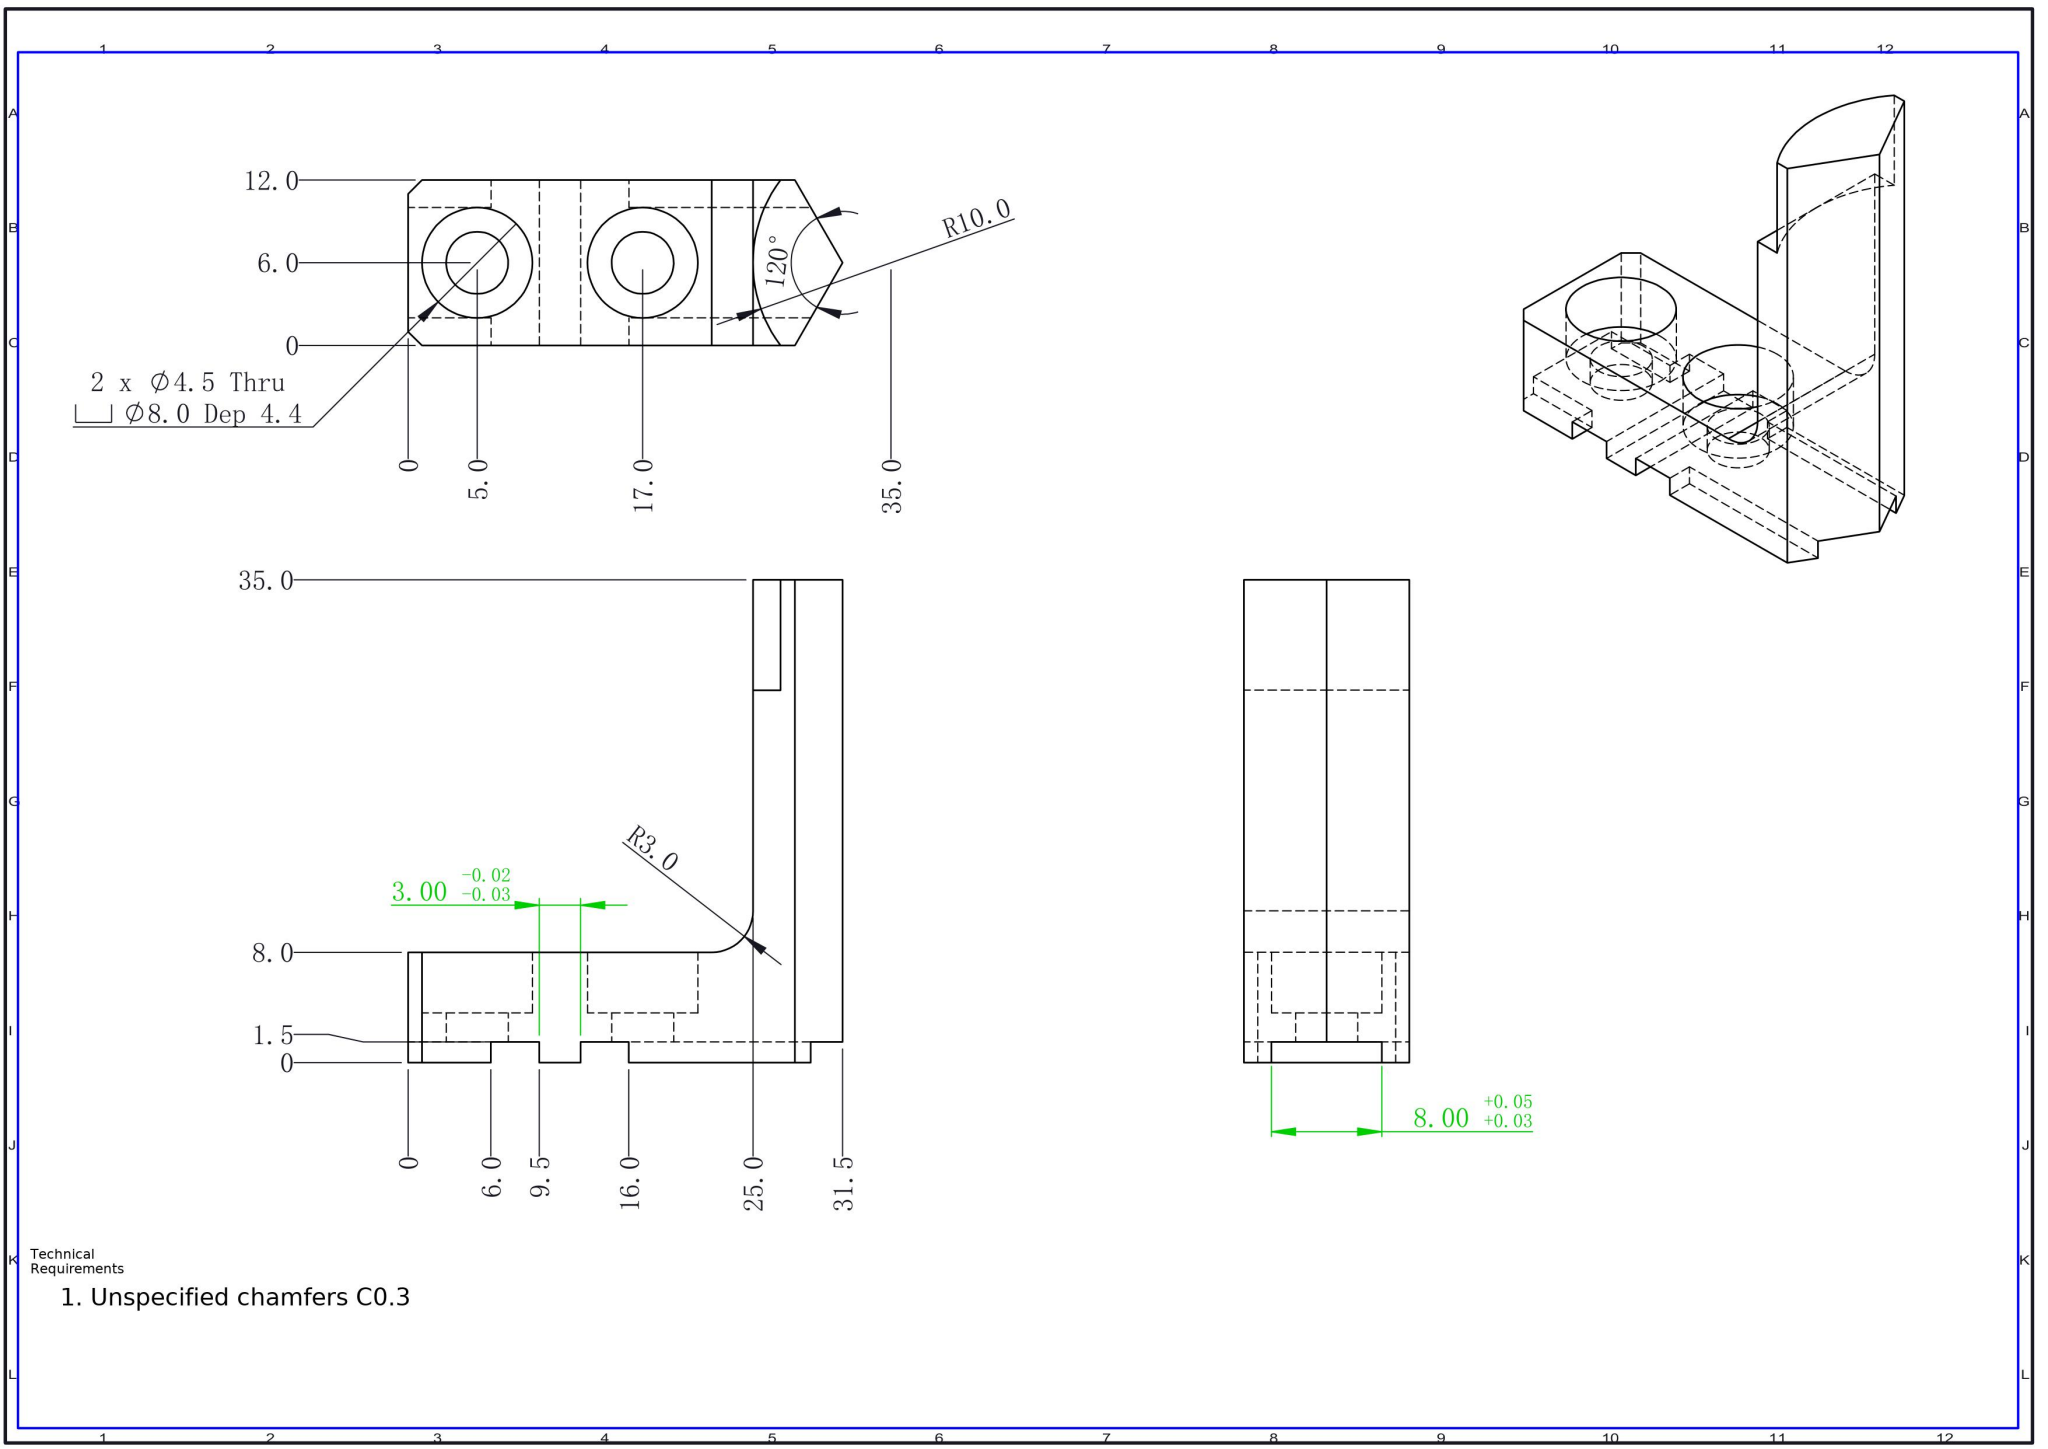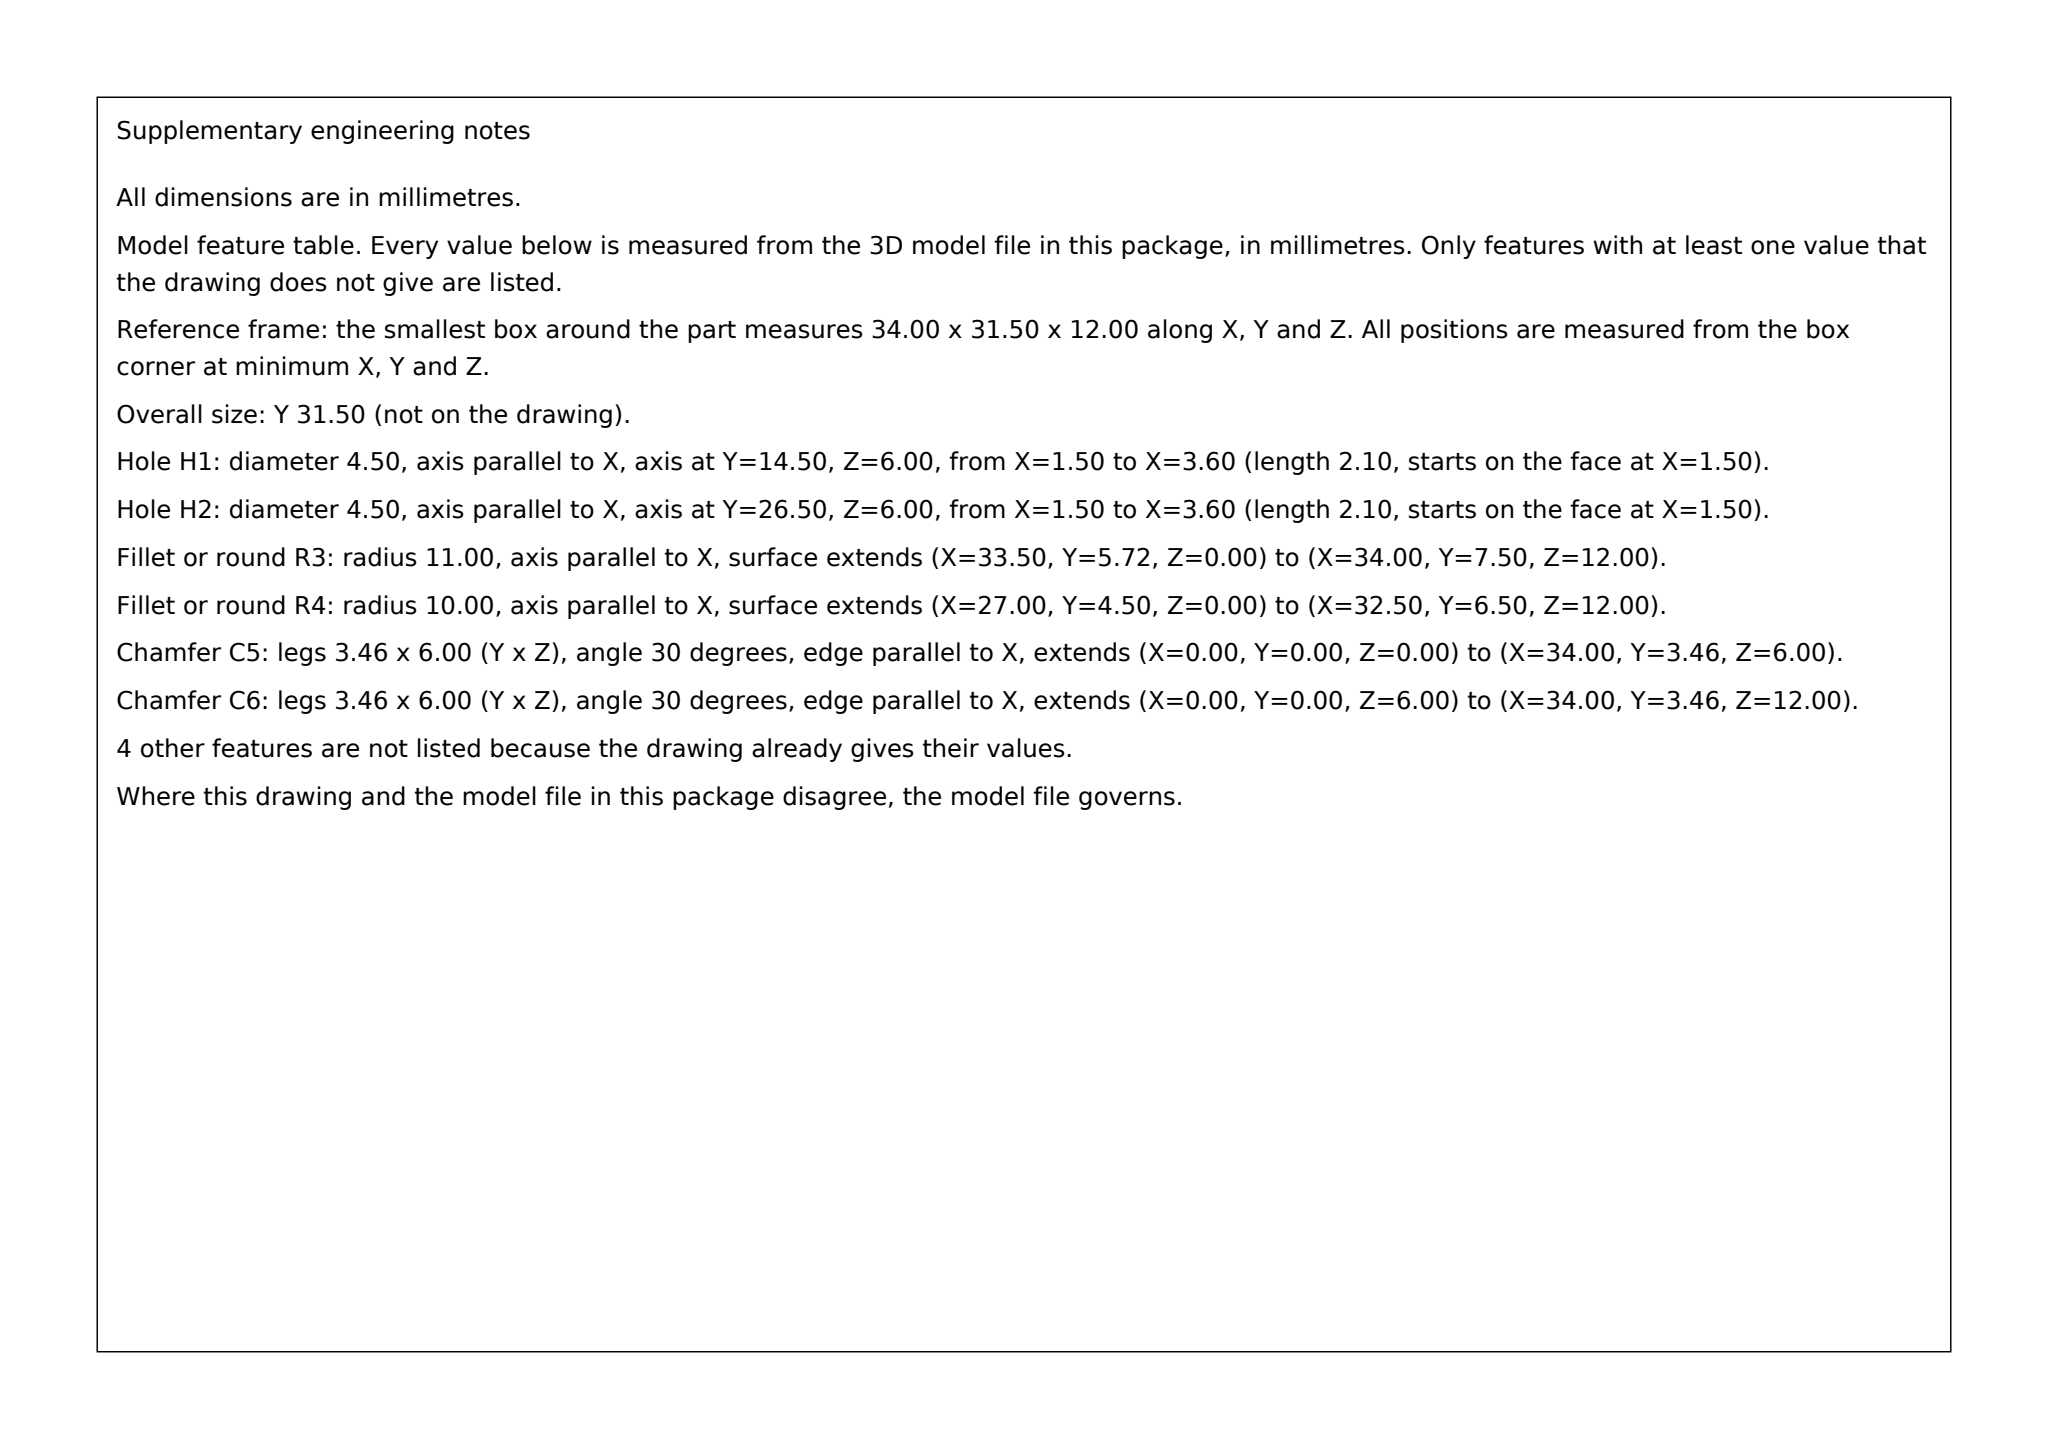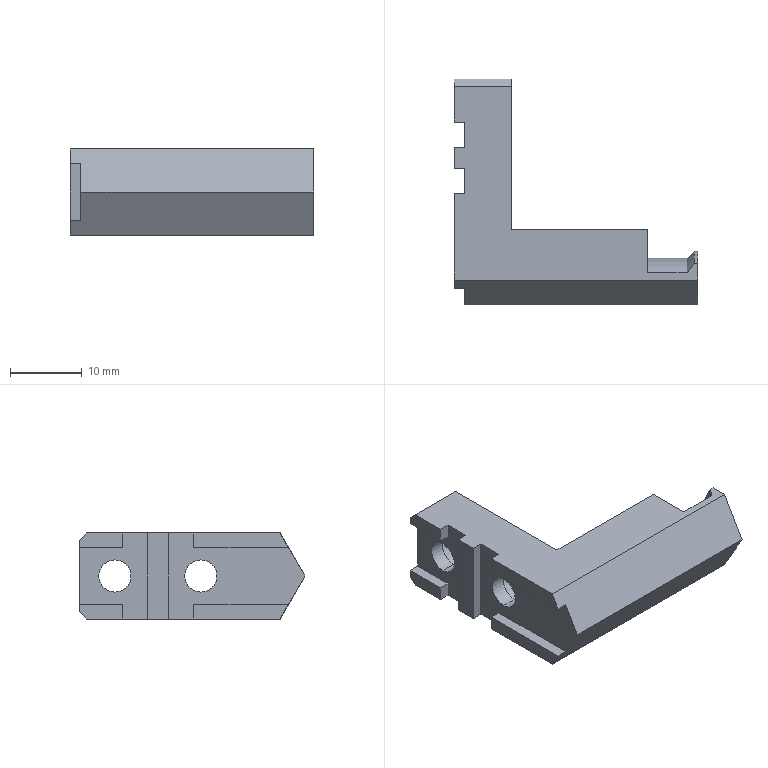Part | SolidWorks | mm | 1 solid | 43 faces | box 34 x 31.5 x 12 mm | volume 4329 mm3 | plane 30 | cylinder 12 | cone 1 | commonest cylinder face diameters 8 x4 4.5 x4 22 x2 20 x2